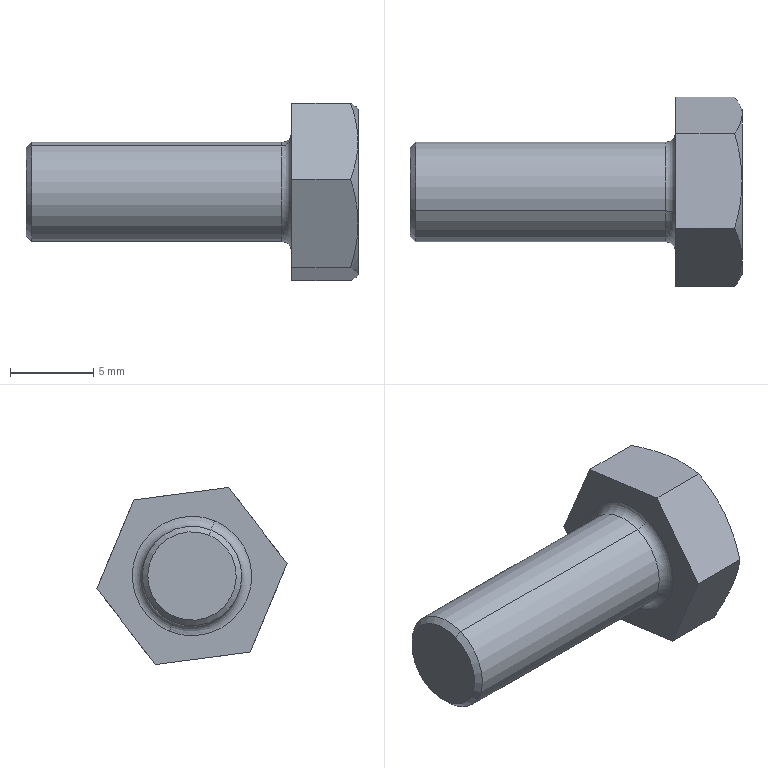Component | NX | HEX_BOLT_M6X16_FT_C | 1 solid | 21 faces | volume 798 mm3 | plane 9 | cone 8 | cylinder 2 | torus 2 | commonest cylinder face diameters 6 x2